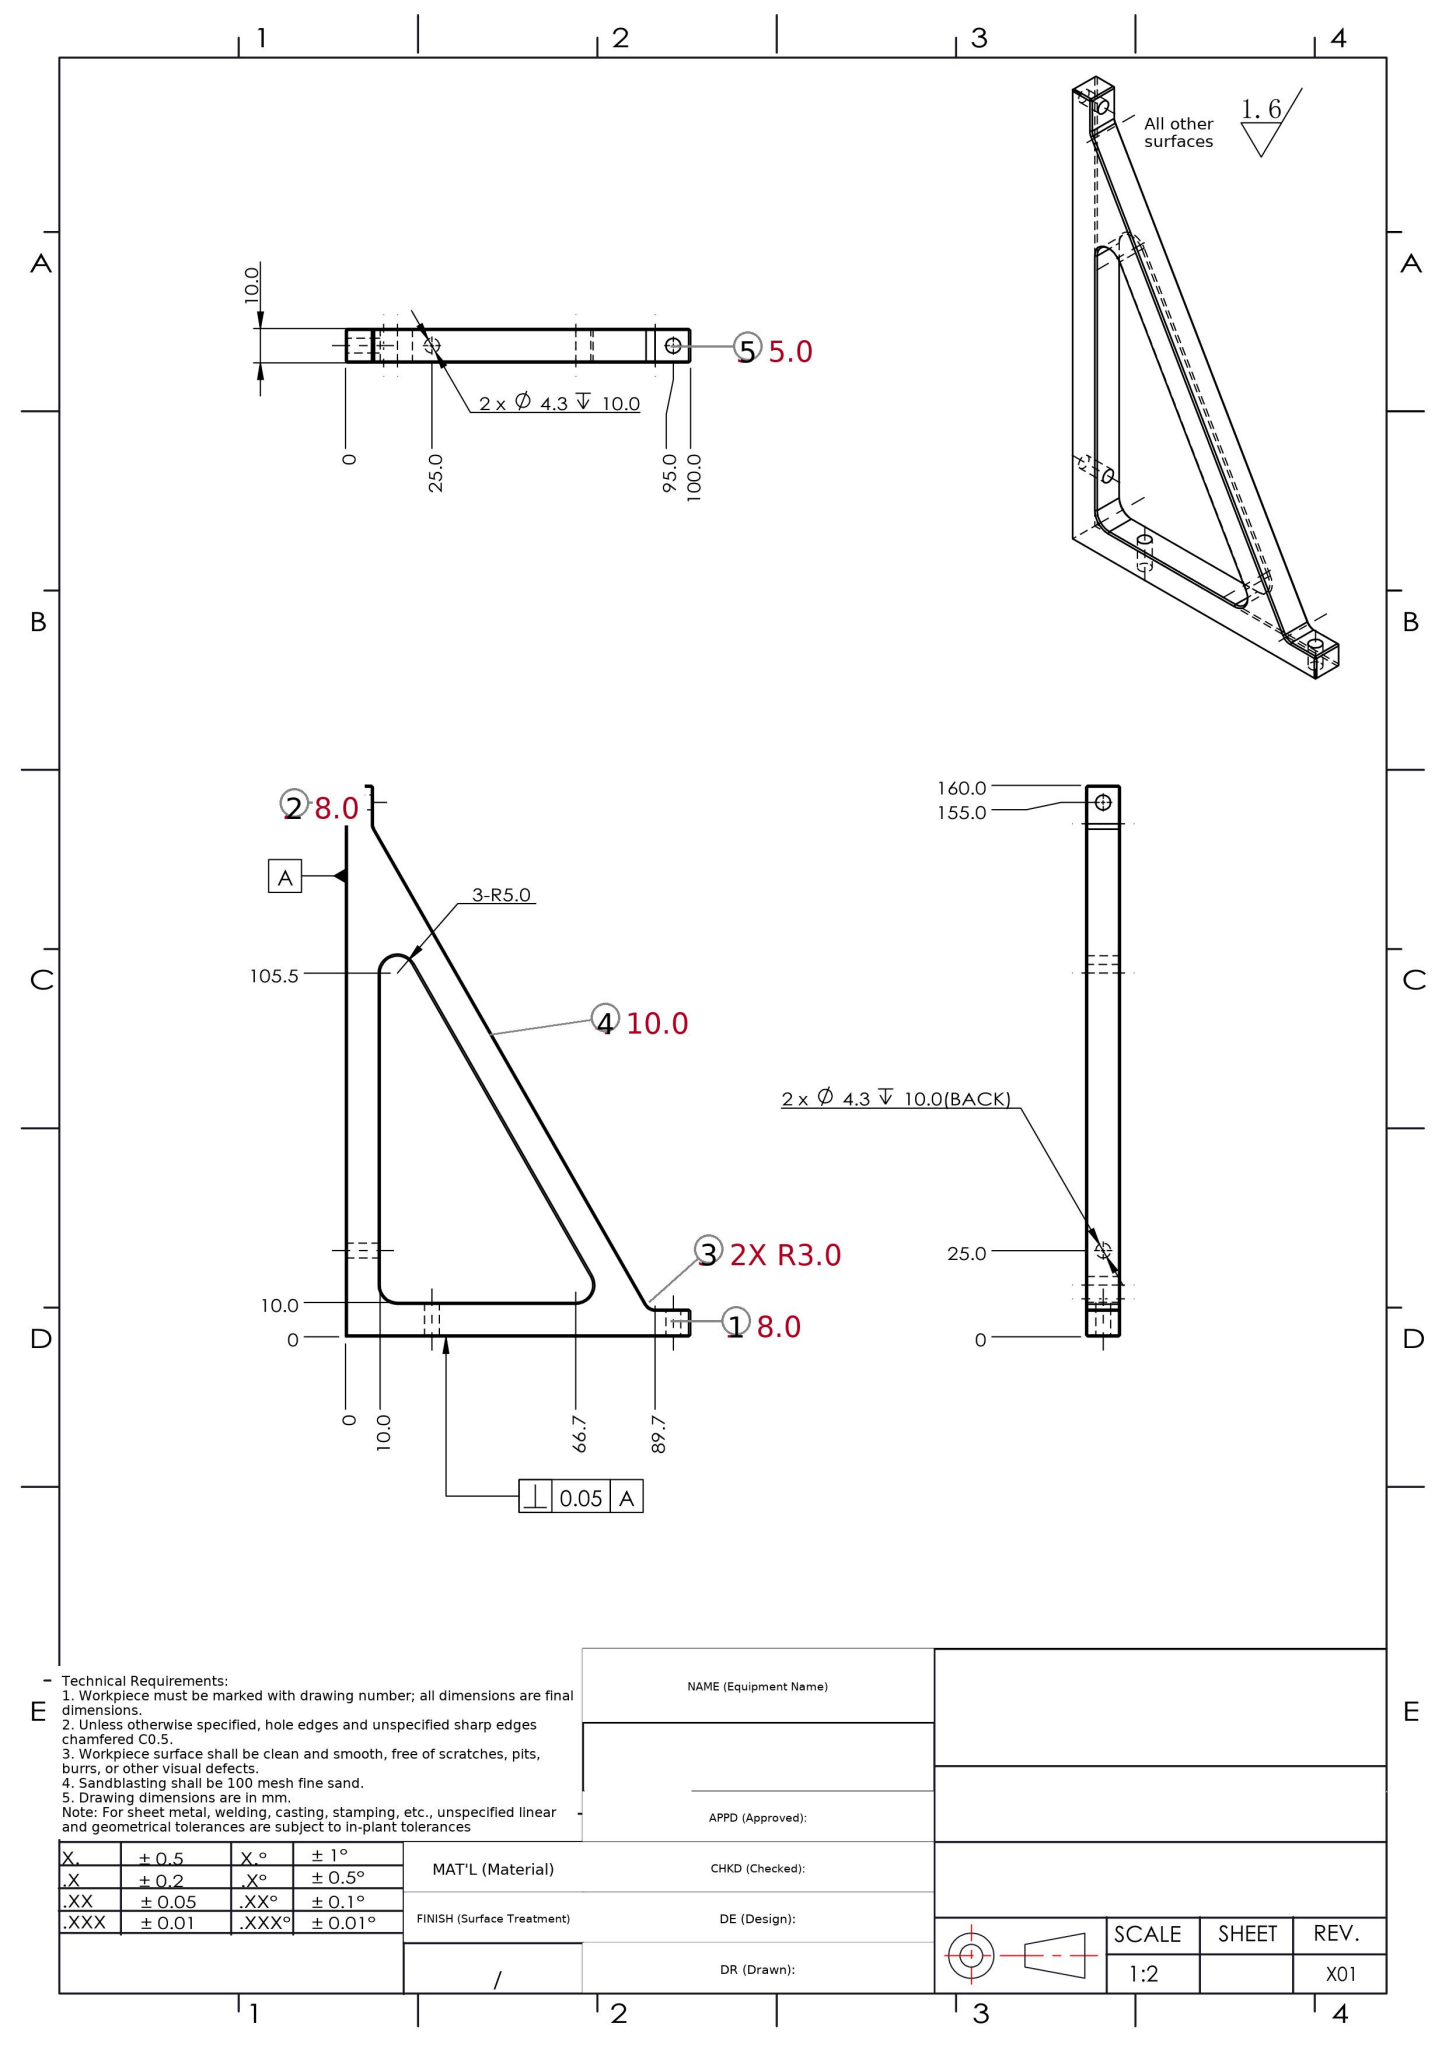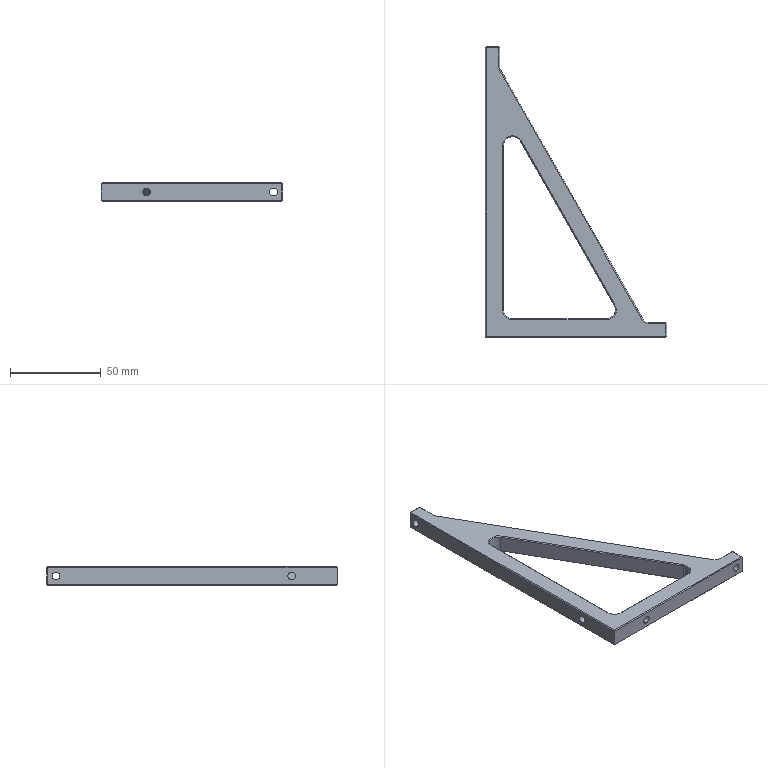Part | SolidWorks | mm | 1 solid | 68 faces | box 100 x 160 x 10 mm | volume 38934 mm3 | plane 44 | cylinder 13 | cone 11 | commonest cylinder face diameters 4.3 x8 10 x3 6 x2
build123d program:
from build123d import *

# Parameters (mm, degrees)
BOSS_EXTRUDE1_DEPTH       = 10
CUT_EXTRUDE1_DEPTH        = 189.944
FILLET1_R                 = 5
M4_CLEARANCE_HOLE1_REACH  = 190.944
M4_CLEARANCE_HOLE1_BORE_R = 2.15
M4_CLEARANCE_HOLE2_REACH  = 190.944
M4_CLEARANCE_HOLE2_BORE_R = 2.15
FILLET2_R                 = 3
CHAMFER1_SIZE             = 0.5


with BuildPart() as part:
    # Sketch1 → Boss-Extrude1 (new body)
    with BuildSketch(Plane.XY):
        Polygon((0, 0), (0, 160), (8, 160), (8, 148), (88, 8), (100, 8), (100, 0), align=None)
    extrude(amount=BOSS_EXTRUDE1_DEPTH)

    # Sketch2 → Cut-Extrude1 (cut, through all)
    with BuildSketch(Plane.XY.offset(10)):
        Polygon((10, 124.344), (10, 10), (75.34, 10), align=None)
    extrude(amount=-CUT_EXTRUDE1_DEPTH, mode=Mode.SUBTRACT)

    # Fillet1
    fillet1_edges = [part.edges().sort_by_distance(p)[0] for p in [
        (10, 124.344, 5),
        (75.34, 10, 5),
        (10, 10, 5),
    ]]
    fillet(fillet1_edges, radius=FILLET1_R)

    # M4 Clearance Hole1 bore → M4 Clearance Hole1 (cut, up to next)
    with BuildSketch(Plane(origin=(0, 0, 0), x_dir=(-1, 0, 0), z_dir=(0, -1, 0)), mode=Mode.PRIVATE) as m4_clearance_hole1_sk1:
        with Locations((-25, -5)):
            Circle(M4_CLEARANCE_HOLE1_BORE_R)
    m4_clearance_hole1_tool1 = extrude(m4_clearance_hole1_sk1.sketch, amount=-M4_CLEARANCE_HOLE1_REACH, mode=Mode.PRIVATE) & part.part
    # M4 Clearance Hole1 bore → M4 Clearance Hole1 (cut, up to next)
    with BuildSketch(Plane(origin=(0, 0, 0), x_dir=(-1, 0, 0), z_dir=(0, -1, 0)), mode=Mode.PRIVATE) as m4_clearance_hole1_sk2:
        with Locations((-95, -5)):
            Circle(M4_CLEARANCE_HOLE1_BORE_R)
    m4_clearance_hole1_tool2 = extrude(m4_clearance_hole1_sk2.sketch, amount=-M4_CLEARANCE_HOLE1_REACH, mode=Mode.PRIVATE) & part.part
    add(m4_clearance_hole1_tool1.solids().sort_by_distance((25, 0, 5))[0], mode=Mode.SUBTRACT)
    add(m4_clearance_hole1_tool2.solids().sort_by_distance((95, 0, 5))[0], mode=Mode.SUBTRACT)

    # M4 Clearance Hole2 bore → M4 Clearance Hole2 (cut, up to next)
    with BuildSketch(Plane.ZY, mode=Mode.PRIVATE) as m4_clearance_hole2_sk1:
        with Locations((5, 25)):
            Circle(M4_CLEARANCE_HOLE2_BORE_R)
    m4_clearance_hole2_tool1 = extrude(m4_clearance_hole2_sk1.sketch, amount=-M4_CLEARANCE_HOLE2_REACH, mode=Mode.PRIVATE) & part.part
    # M4 Clearance Hole2 bore → M4 Clearance Hole2 (cut, up to next)
    with BuildSketch(Plane.ZY, mode=Mode.PRIVATE) as m4_clearance_hole2_sk2:
        with Locations((5, 155)):
            Circle(M4_CLEARANCE_HOLE2_BORE_R)
    m4_clearance_hole2_tool2 = extrude(m4_clearance_hole2_sk2.sketch, amount=-M4_CLEARANCE_HOLE2_REACH, mode=Mode.PRIVATE) & part.part
    add(m4_clearance_hole2_tool1.solids().sort_by_distance((0, 25, 5))[0], mode=Mode.SUBTRACT)
    add(m4_clearance_hole2_tool2.solids().sort_by_distance((0, 155, 5))[0], mode=Mode.SUBTRACT)

    # Fillet2
    fillet2_edges = [part.edges().sort_by_distance(p)[0] for p in [
        (8, 148, 5),
        (88, 8, 5),
    ]]
    fillet(fillet2_edges, radius=FILLET2_R)

    # Chamfer1
    chamfer1_edges = [part.edges().sort_by_distance(p)[0] for p in [
        (94.87, 8, 10),
        (0, 160, 5),
        (8, 160, 5),
        (100, 8, 5),
        (100, 0, 5),
        (4, 160, 10),
        (0, 80, 10),
        (40.862, 10, 10),
        (40.862, 10, 0),
        (10, 60.258, 10),
        (10, 60.258, 0),
        (45.203, 62.739, 10),
        (45.203, 62.739, 0),
        (11.464, 11.464, 10),
        (50, 0, 10),
        (11.464, 11.464, 0),
        (13.717, 110.349, 10),
        (13.717, 110.349, 0),
        (71.048, 12.49, 10),
        (71.048, 12.49, 0),
        (0, 80, 0),
        (100, 4, 10),
        (4, 160, 0),
        (47.766, 78.41, 0),
        (47.766, 78.41, 10),
        (8, 154.398, 0),
        (8, 154.398, 10),
        (88.235, 8.405, 0),
        (88.235, 8.405, 10),
        (8.101, 148.027, 0),
        (8.101, 148.027, 10),
        (94.87, 8, 0),
        (100, 4, 0),
        (50, 0, 0),
    ]]
    chamfer(chamfer1_edges, length=CHAMFER1_SIZE)


solid = part.part